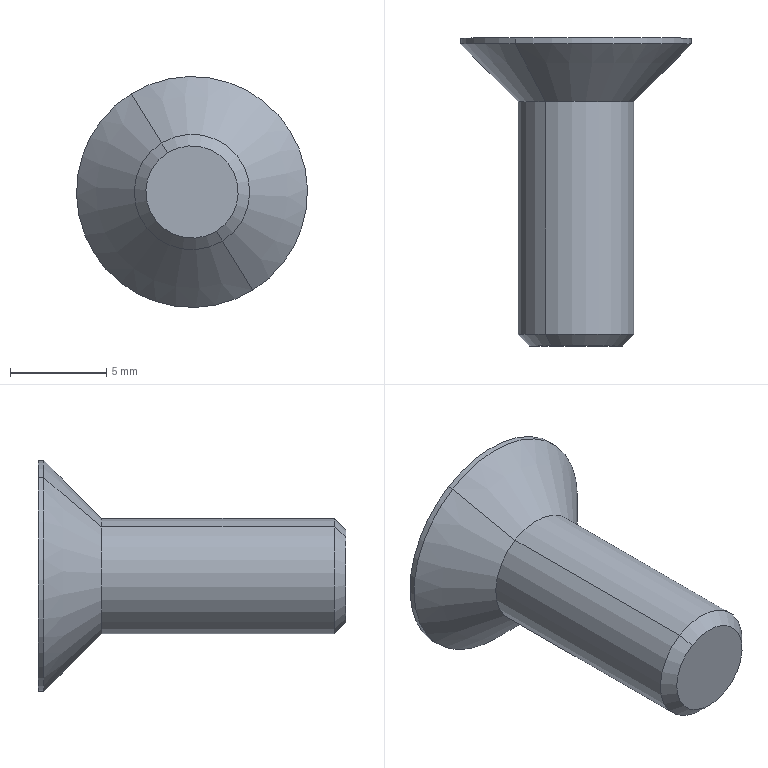Component | SolidWorks | 2012MB0201-1_UpperRackCoverModule-1_HexSocketFlatHeadScrewM6-16FerrousOxide-12 | 1 solid | 24 faces | box 12 x 16 x 12 mm | volume 549 mm3 | plane 14 | cone 6 | cylinder 4 | commonest cylinder face diameters 6 x2 12 x2 | material SCM435
STEP:
#1=COLOUR_RGB('',0.7922,0.8196,0.9333);
#2=FILL_AREA_STYLE_COLOUR('',#1);
#3=FILL_AREA_STYLE('',(#2));
#4=SURFACE_STYLE_FILL_AREA(#3);
#5=SURFACE_SIDE_STYLE('',(#4));
#6=SURFACE_STYLE_USAGE(.BOTH.,#5);
#7=PRESENTATION_STYLE_ASSIGNMENT((#6));
#8=CARTESIAN_POINT('',(-69.541,40.663,-12.118));
#9=VERTEX_POINT('',#8);
#10=CARTESIAN_POINT('',(-69.441,40.663,-12.278));
#11=VERTEX_POINT('',#10);
#12=CARTESIAN_POINT('',(-69.491,40.663,-12.198));
#13=DIRECTION('',(0.,-1.,-0.));
#14=DIRECTION('',(0.8493,0.,0.5279));
#15=AXIS2_PLACEMENT_3D('',#12,#13,#14);
#16=CIRCLE('',#15,0.09449);
#17=EDGE_CURVE('',#9,#11,#16,.T.);
#18=ORIENTED_EDGE('',*,*,#17,.F.);
#19=CARTESIAN_POINT('',(-69.553,40.687,-12.097));
#20=VERTEX_POINT('',#19);
#21=CARTESIAN_POINT('',(-69.541,40.663,-12.118));
#22=DIRECTION('',(-0.3733,0.7071,0.6005));
#23=VECTOR('',#22,39.37);
#24=LINE('',#21,#23);
#25=EDGE_CURVE('',#9,#20,#24,.T.);
#26=ORIENTED_EDGE('',*,*,#25,.T.);
#27=CARTESIAN_POINT('',(-69.429,40.687,-12.298));
#28=VERTEX_POINT('',#27);
#29=CARTESIAN_POINT('',(-69.491,40.687,-12.198));
#30=DIRECTION('',(-0.,1.,0.));
#31=DIRECTION('',(0.5279,0.,-0.8493));
#32=AXIS2_PLACEMENT_3D('',#29,#30,#31);
#33=CIRCLE('',#32,0.1181);
#34=EDGE_CURVE('',#28,#20,#33,.T.);
#35=ORIENTED_EDGE('',*,*,#34,.F.);
#36=CARTESIAN_POINT('',(-69.441,40.663,-12.278));
#37=DIRECTION('',(0.3733,0.7071,-0.6005));
#38=VECTOR('',#37,39.37);
#39=LINE('',#36,#38);
#40=EDGE_CURVE('',#11,#28,#39,.T.);
#41=ORIENTED_EDGE('',*,*,#40,.F.);
#42=EDGE_LOOP('',(#18,#26,#35,#41));
#43=FACE_OUTER_BOUND('',#42,.T.);
#44=CARTESIAN_POINT('',(-69.491,40.663,-12.198));
#45=DIRECTION('',(-0.,1.,0.));
#46=DIRECTION('',(0.5279,0.,-0.8493));
#47=AXIS2_PLACEMENT_3D('',#44,#45,#46);
#48=CONICAL_SURFACE('',#47,0.09449,0.7854);
#49=ADVANCED_FACE('',(#43),#48,.T.);
#50=ORIENTED_EDGE('',*,*,#34,.T.);
#51=CARTESIAN_POINT('',(-69.553,41.163,-12.097));
#52=VERTEX_POINT('',#51);
#53=CARTESIAN_POINT('',(-69.553,39.719,-12.097));
#54=DIRECTION('',(-0.,1.,0.));
#55=VECTOR('',#54,39.37);
#56=LINE('',#53,#55);
#57=EDGE_CURVE('',#20,#52,#56,.T.);
#58=ORIENTED_EDGE('',*,*,#57,.T.);
#59=CARTESIAN_POINT('',(-69.429,41.163,-12.298));
#60=VERTEX_POINT('',#59);
#61=CARTESIAN_POINT('',(-69.491,41.163,-12.198));
#62=DIRECTION('',(0.,-1.,-0.));
#63=DIRECTION('',(0.5279,0.,-0.8493));
#64=AXIS2_PLACEMENT_3D('',#61,#62,#63);
#65=CIRCLE('',#64,0.1181);
#66=EDGE_CURVE('',#52,#60,#65,.T.);
#67=ORIENTED_EDGE('',*,*,#66,.T.);
#68=CARTESIAN_POINT('',(-69.429,39.719,-12.298));
#69=DIRECTION('',(-0.,1.,0.));
#70=VECTOR('',#69,39.37);
#71=LINE('',#68,#70);
#72=EDGE_CURVE('',#28,#60,#71,.T.);
#73=ORIENTED_EDGE('',*,*,#72,.F.);
#74=EDGE_LOOP('',(#50,#58,#67,#73));
#75=FACE_OUTER_BOUND('',#74,.T.);
#76=CARTESIAN_POINT('',(-69.491,39.719,-12.198));
#77=DIRECTION('',(-0.,1.,0.));
#78=DIRECTION('',(0.5279,0.,-0.8493));
#79=AXIS2_PLACEMENT_3D('',#76,#77,#78);
#80=CYLINDRICAL_SURFACE('',#79,0.1181);
#81=ADVANCED_FACE('',(#75),#80,.T.);
#82=ORIENTED_EDGE('',*,*,#66,.F.);
#83=CARTESIAN_POINT('',(-69.616,41.282,-11.997));
#84=VERTEX_POINT('',#83);
#85=CARTESIAN_POINT('',(-69.616,41.282,-11.997));
#86=DIRECTION('',(-0.3733,0.7071,0.6005));
#87=VECTOR('',#86,39.37);
#88=LINE('',#85,#87);
#89=EDGE_CURVE('',#52,#84,#88,.T.);
#90=ORIENTED_EDGE('',*,*,#89,.T.);
#91=CARTESIAN_POINT('',(-69.366,41.282,-12.398));
#92=VERTEX_POINT('',#91);
#93=CARTESIAN_POINT('',(-69.491,41.282,-12.198));
#94=DIRECTION('',(0.,-1.,-0.));
#95=DIRECTION('',(0.5279,0.,-0.8493));
#96=AXIS2_PLACEMENT_3D('',#93,#94,#95);
#97=CIRCLE('',#96,0.2362);
#98=EDGE_CURVE('',#84,#92,#97,.T.);
#99=ORIENTED_EDGE('',*,*,#98,.T.);
#100=CARTESIAN_POINT('',(-69.366,41.282,-12.398));
#101=DIRECTION('',(0.3733,0.7071,-0.6005));
#102=VECTOR('',#101,39.37);
#103=LINE('',#100,#102);
#104=EDGE_CURVE('',#60,#92,#103,.T.);
#105=ORIENTED_EDGE('',*,*,#104,.F.);
#106=EDGE_LOOP('',(#82,#90,#99,#105));
#107=FACE_OUTER_BOUND('',#106,.T.);
#108=CARTESIAN_POINT('',(-69.491,41.282,-12.198));
#109=DIRECTION('',(-0.,1.,0.));
#110=DIRECTION('',(0.5279,0.,-0.8493));
#111=AXIS2_PLACEMENT_3D('',#108,#109,#110);
#112=CONICAL_SURFACE('',#111,0.2362,0.7854);
#113=ADVANCED_FACE('',(#107),#112,.T.);
#114=ORIENTED_EDGE('',*,*,#98,.F.);
#115=CARTESIAN_POINT('',(-69.616,41.293,-11.997));
#116=VERTEX_POINT('',#115);
#117=CARTESIAN_POINT('',(-69.616,39.719,-11.997));
#118=DIRECTION('',(-0.,1.,0.));
#119=VECTOR('',#118,39.37);
#120=LINE('',#117,#119);
#121=EDGE_CURVE('',#84,#116,#120,.T.);
#122=ORIENTED_EDGE('',*,*,#121,.T.);
#123=CARTESIAN_POINT('',(-69.366,41.293,-12.398));
#124=VERTEX_POINT('',#123);
#125=CARTESIAN_POINT('',(-69.491,41.293,-12.198));
#126=DIRECTION('',(0.,-1.,-0.));
#127=DIRECTION('',(0.5279,0.,-0.8493));
#128=AXIS2_PLACEMENT_3D('',#125,#126,#127);
#129=CIRCLE('',#128,0.2362);
#130=EDGE_CURVE('',#116,#124,#129,.T.);
#131=ORIENTED_EDGE('',*,*,#130,.T.);
#132=CARTESIAN_POINT('',(-69.366,39.719,-12.398));
#133=DIRECTION('',(-0.,1.,0.));
#134=VECTOR('',#133,39.37);
#135=LINE('',#132,#134);
#136=EDGE_CURVE('',#92,#124,#135,.T.);
#137=ORIENTED_EDGE('',*,*,#136,.F.);
#138=EDGE_LOOP('',(#114,#122,#131,#137));
#139=FACE_OUTER_BOUND('',#138,.T.);
#140=CARTESIAN_POINT('',(-69.491,39.719,-12.198));
#141=DIRECTION('',(-0.,1.,0.));
#142=DIRECTION('',(0.5279,0.,-0.8493));
#143=AXIS2_PLACEMENT_3D('',#140,#141,#142);
#144=CYLINDRICAL_SURFACE('',#143,0.2362);
#145=ADVANCED_FACE('',(#139),#144,.T.);
#146=CARTESIAN_POINT('',(-69.491,41.168,-12.198));
#147=VERTEX_POINT('',#146);
#148=CARTESIAN_POINT('',(-69.449,41.189,-12.265));
#149=VERTEX_POINT('',#148);
#150=CARTESIAN_POINT('',(-69.449,41.189,-12.265));
#151=DIRECTION('',(0.5099,0.2588,-0.8204));
#152=VECTOR('',#151,39.37);
#153=LINE('',#150,#152);
#154=EDGE_CURVE('',#147,#149,#153,.T.);
#155=ORIENTED_EDGE('',*,*,#154,.F.);
#156=CARTESIAN_POINT('',(-69.532,41.189,-12.131));
#157=VERTEX_POINT('',#156);
#158=CARTESIAN_POINT('',(-69.532,41.189,-12.131));
#159=DIRECTION('',(-0.5099,0.2588,0.8204));
#160=VECTOR('',#159,39.37);
#161=LINE('',#158,#160);
#162=EDGE_CURVE('',#147,#157,#161,.T.);
#163=ORIENTED_EDGE('',*,*,#162,.T.);
#164=CARTESIAN_POINT('',(-69.454,41.189,-12.128));
#165=VERTEX_POINT('',#164);
#166=CARTESIAN_POINT('',(-69.491,41.189,-12.198));
#167=DIRECTION('',(0.,-1.,-0.));
#168=DIRECTION('',(0.5279,0.,-0.8493));
#169=AXIS2_PLACEMENT_3D('',#166,#167,#168);
#170=CIRCLE('',#169,0.07874);
#171=EDGE_CURVE('',#165,#157,#170,.T.);
#172=ORIENTED_EDGE('',*,*,#171,.F.);
#173=CARTESIAN_POINT('',(-69.412,41.189,-12.195));
#174=VERTEX_POINT('',#173);
#175=CARTESIAN_POINT('',(-69.491,41.189,-12.198));
#176=DIRECTION('',(0.,-1.,-0.));
#177=DIRECTION('',(0.5279,0.,-0.8493));
#178=AXIS2_PLACEMENT_3D('',#175,#176,#177);
#179=CIRCLE('',#178,0.07874);
#180=EDGE_CURVE('',#174,#165,#179,.T.);
#181=ORIENTED_EDGE('',*,*,#180,.F.);
#182=CARTESIAN_POINT('',(-69.491,41.189,-12.198));
#183=DIRECTION('',(0.,-1.,-0.));
#184=DIRECTION('',(0.5279,0.,-0.8493));
#185=AXIS2_PLACEMENT_3D('',#182,#183,#184);
#186=CIRCLE('',#185,0.07874);
#187=EDGE_CURVE('',#149,#174,#186,.T.);
#188=ORIENTED_EDGE('',*,*,#187,.F.);
#189=EDGE_LOOP('',(#155,#163,#172,#181,#188));
#190=FACE_OUTER_BOUND('',#189,.T.);
#191=CARTESIAN_POINT('',(-69.491,41.189,-12.198));
#192=DIRECTION('',(-0.,1.,0.));
#193=DIRECTION('',(0.5279,0.,-0.8493));
#194=AXIS2_PLACEMENT_3D('',#191,#192,#193);
#195=CONICAL_SURFACE('',#194,0.07874,1.309);
#196=ADVANCED_FACE('',(#190),#195,.F.);
#197=ORIENTED_EDGE('',*,*,#57,.F.);
#198=CARTESIAN_POINT('',(-69.491,40.687,-12.198));
#199=DIRECTION('',(-0.,1.,0.));
#200=DIRECTION('',(0.5279,0.,-0.8493));
#201=AXIS2_PLACEMENT_3D('',#198,#199,#200);
#202=CIRCLE('',#201,0.1181);
#203=EDGE_CURVE('',#20,#28,#202,.T.);
#204=ORIENTED_EDGE('',*,*,#203,.T.);
#205=ORIENTED_EDGE('',*,*,#72,.T.);
#206=CARTESIAN_POINT('',(-69.491,41.163,-12.198));
#207=DIRECTION('',(0.,-1.,-0.));
#208=DIRECTION('',(0.5279,0.,-0.8493));
#209=AXIS2_PLACEMENT_3D('',#206,#207,#208);
#210=CIRCLE('',#209,0.1181);
#211=EDGE_CURVE('',#60,#52,#210,.T.);
#212=ORIENTED_EDGE('',*,*,#211,.T.);
#213=EDGE_LOOP('',(#197,#204,#205,#212));
#214=FACE_OUTER_BOUND('',#213,.T.);
#215=CARTESIAN_POINT('',(-69.491,39.719,-12.198));
#216=DIRECTION('',(-0.,1.,0.));
#217=DIRECTION('',(0.5279,0.,-0.8493));
#218=AXIS2_PLACEMENT_3D('',#215,#216,#217);
#219=CYLINDRICAL_SURFACE('',#218,0.1181);
#220=ADVANCED_FACE('',(#214),#219,.T.);
#221=ORIENTED_EDGE('',*,*,#89,.F.);
#222=ORIENTED_EDGE('',*,*,#211,.F.);
#223=ORIENTED_EDGE('',*,*,#104,.T.);
#224=CARTESIAN_POINT('',(-69.491,41.282,-12.198));
#225=DIRECTION('',(0.,-1.,-0.));
#226=DIRECTION('',(0.5279,0.,-0.8493));
#227=AXIS2_PLACEMENT_3D('',#224,#225,#226);
#228=CIRCLE('',#227,0.2362);
#229=EDGE_CURVE('',#92,#84,#228,.T.);
#230=ORIENTED_EDGE('',*,*,#229,.T.);
#231=EDGE_LOOP('',(#221,#222,#223,#230));
#232=FACE_OUTER_BOUND('',#231,.T.);
#233=CARTESIAN_POINT('',(-69.491,41.282,-12.198));
#234=DIRECTION('',(-0.,1.,0.));
#235=DIRECTION('',(0.5279,0.,-0.8493));
#236=AXIS2_PLACEMENT_3D('',#233,#234,#235);
#237=CONICAL_SURFACE('',#236,0.2362,0.7854);
#238=ADVANCED_FACE('',(#232),#237,.T.);
#239=ORIENTED_EDGE('',*,*,#121,.F.);
#240=ORIENTED_EDGE('',*,*,#229,.F.);
#241=ORIENTED_EDGE('',*,*,#136,.T.);
#242=CARTESIAN_POINT('',(-69.491,41.293,-12.198));
#243=DIRECTION('',(0.,-1.,-0.));
#244=DIRECTION('',(0.5279,0.,-0.8493));
#245=AXIS2_PLACEMENT_3D('',#242,#243,#244);
#246=CIRCLE('',#245,0.2362);
#247=EDGE_CURVE('',#124,#116,#246,.T.);
#248=ORIENTED_EDGE('',*,*,#247,.T.);
#249=EDGE_LOOP('',(#239,#240,#241,#248));
#250=FACE_OUTER_BOUND('',#249,.T.);
#251=CARTESIAN_POINT('',(-69.491,39.719,-12.198));
#252=DIRECTION('',(-0.,1.,0.));
#253=DIRECTION('',(0.5279,0.,-0.8493));
#254=AXIS2_PLACEMENT_3D('',#251,#252,#253);
#255=CYLINDRICAL_SURFACE('',#254,0.2362);
#256=ADVANCED_FACE('',(#250),#255,.T.);
#257=CARTESIAN_POINT('',(-69.494,41.293,-12.107));
#258=VERTEX_POINT('',#257);
#259=CARTESIAN_POINT('',(-69.414,41.293,-12.15));
#260=VERTEX_POINT('',#259);
#261=CARTESIAN_POINT('',(-69.494,41.293,-12.107));
#262=DIRECTION('',(0.8818,0.,-0.4716));
#263=VECTOR('',#262,39.37);
#264=LINE('',#261,#263);
#265=EDGE_CURVE('',#258,#260,#264,.T.);
#266=ORIENTED_EDGE('',*,*,#265,.F.);
#267=CARTESIAN_POINT('',(-69.571,41.293,-12.155));
#268=VERTEX_POINT('',#267);
#269=CARTESIAN_POINT('',(-69.532,41.293,-12.131));
#270=DIRECTION('',(0.8493,0.,0.5279));
#271=VECTOR('',#270,39.37);
#272=LINE('',#269,#271);
#273=EDGE_CURVE('',#268,#258,#272,.T.);
#274=ORIENTED_EDGE('',*,*,#273,.F.);
#275=CARTESIAN_POINT('',(-69.568,41.293,-12.246));
#276=VERTEX_POINT('',#275);
#277=CARTESIAN_POINT('',(-69.568,41.293,-12.246));
#278=DIRECTION('',(-0.03252,-0.,0.9995));
#279=VECTOR('',#278,39.37);
#280=LINE('',#277,#279);
#281=EDGE_CURVE('',#276,#268,#280,.T.);
#282=ORIENTED_EDGE('',*,*,#281,.F.);
#283=CARTESIAN_POINT('',(-69.488,41.293,-12.289));
#284=VERTEX_POINT('',#283);
#285=CARTESIAN_POINT('',(-69.488,41.293,-12.289));
#286=DIRECTION('',(-0.8818,-0.,0.4716));
#287=VECTOR('',#286,39.37);
#288=LINE('',#285,#287);
#289=EDGE_CURVE('',#284,#276,#288,.T.);
#290=ORIENTED_EDGE('',*,*,#289,.F.);
#291=CARTESIAN_POINT('',(-69.411,41.293,-12.241));
#292=VERTEX_POINT('',#291);
#293=CARTESIAN_POINT('',(-69.449,41.293,-12.265));
#294=DIRECTION('',(-0.8493,-0.,-0.5279));
#295=VECTOR('',#294,39.37);
#296=LINE('',#293,#295);
#297=EDGE_CURVE('',#292,#284,#296,.T.);
#298=ORIENTED_EDGE('',*,*,#297,.F.);
#299=CARTESIAN_POINT('',(-69.414,41.293,-12.15));
#300=DIRECTION('',(0.03252,0.,-0.9995));
#301=VECTOR('',#300,39.37);
#302=LINE('',#299,#301);
#303=EDGE_CURVE('',#260,#292,#302,.T.);
#304=ORIENTED_EDGE('',*,*,#303,.F.);
#305=EDGE_LOOP('',(#266,#274,#282,#290,#298,#304));
#306=FACE_BOUND('',#305,.T.);
#307=ORIENTED_EDGE('',*,*,#247,.F.);
#308=ORIENTED_EDGE('',*,*,#130,.F.);
#309=EDGE_LOOP('',(#307,#308));
#310=FACE_OUTER_BOUND('',#309,.T.);
#311=CARTESIAN_POINT('',(-69.491,41.293,-12.198));
#312=DIRECTION('',(0.,-1.,-0.));
#313=DIRECTION('',(-0.5279,-0.,0.8493));
#314=AXIS2_PLACEMENT_3D('',#311,#312,#313);
#315=PLANE('',#314);
#316=ADVANCED_FACE('',(#306,#310),#315,.F.);
#317=CARTESIAN_POINT('',(-69.414,41.189,-12.15));
#318=VERTEX_POINT('',#317);
#319=CARTESIAN_POINT('',(-69.412,41.189,-12.195));
#320=DIRECTION('',(-0.03252,-0.,0.9995));
#321=VECTOR('',#320,39.37);
#322=LINE('',#319,#321);
#323=EDGE_CURVE('',#174,#318,#322,.T.);
#324=ORIENTED_EDGE('',*,*,#323,.T.);
#325=CARTESIAN_POINT('',(-69.414,41.189,-12.15));
#326=DIRECTION('',(-0.,1.,0.));
#327=VECTOR('',#326,39.37);
#328=LINE('',#325,#327);
#329=EDGE_CURVE('',#318,#260,#328,.T.);
#330=ORIENTED_EDGE('',*,*,#329,.T.);
#331=ORIENTED_EDGE('',*,*,#303,.T.);
#332=CARTESIAN_POINT('',(-69.411,41.189,-12.241));
#333=VERTEX_POINT('',#332);
#334=CARTESIAN_POINT('',(-69.411,41.189,-12.241));
#335=DIRECTION('',(0.,-1.,-0.));
#336=VECTOR('',#335,39.37);
#337=LINE('',#334,#336);
#338=EDGE_CURVE('',#292,#333,#337,.T.);
#339=ORIENTED_EDGE('',*,*,#338,.T.);
#340=CARTESIAN_POINT('',(-69.411,41.189,-12.241));
#341=DIRECTION('',(-0.03252,-0.,0.9995));
#342=VECTOR('',#341,39.37);
#343=LINE('',#340,#342);
#344=EDGE_CURVE('',#333,#174,#343,.T.);
#345=ORIENTED_EDGE('',*,*,#344,.T.);
#346=EDGE_LOOP('',(#324,#330,#331,#339,#345));
#347=FACE_OUTER_BOUND('',#346,.T.);
#348=CARTESIAN_POINT('',(-69.411,41.189,-12.241));
#349=DIRECTION('',(-0.9995,-0.,-0.03252));
#350=DIRECTION('',(0.03252,0.,-0.9995));
#351=AXIS2_PLACEMENT_3D('',#348,#349,#350);
#352=PLANE('',#351);
#353=ADVANCED_FACE('',(#347),#352,.T.);
#354=CARTESIAN_POINT('',(-69.494,41.189,-12.107));
#355=VERTEX_POINT('',#354);
#356=CARTESIAN_POINT('',(-69.454,41.189,-12.128));
#357=DIRECTION('',(-0.8818,-0.,0.4716));
#358=VECTOR('',#357,39.37);
#359=LINE('',#356,#358);
#360=EDGE_CURVE('',#165,#355,#359,.T.);
#361=ORIENTED_EDGE('',*,*,#360,.T.);
#362=CARTESIAN_POINT('',(-69.494,41.189,-12.107));
#363=DIRECTION('',(-0.,1.,0.));
#364=VECTOR('',#363,39.37);
#365=LINE('',#362,#364);
#366=EDGE_CURVE('',#355,#258,#365,.T.);
#367=ORIENTED_EDGE('',*,*,#366,.T.);
#368=ORIENTED_EDGE('',*,*,#265,.T.);
#369=ORIENTED_EDGE('',*,*,#329,.F.);
#370=CARTESIAN_POINT('',(-69.414,41.189,-12.15));
#371=DIRECTION('',(-0.8818,-0.,0.4716));
#372=VECTOR('',#371,39.37);
#373=LINE('',#370,#372);
#374=EDGE_CURVE('',#318,#165,#373,.T.);
#375=ORIENTED_EDGE('',*,*,#374,.T.);
#376=EDGE_LOOP('',(#361,#367,#368,#369,#375));
#377=FACE_OUTER_BOUND('',#376,.T.);
#378=CARTESIAN_POINT('',(-69.414,41.189,-12.15));
#379=DIRECTION('',(-0.4716,-0.,-0.8818));
#380=DIRECTION('',(0.8818,0.,-0.4716));
#381=AXIS2_PLACEMENT_3D('',#378,#379,#380);
#382=PLANE('',#381);
#383=ADVANCED_FACE('',(#377),#382,.T.);
#384=CARTESIAN_POINT('',(-69.571,41.189,-12.155));
#385=VERTEX_POINT('',#384);
#386=CARTESIAN_POINT('',(-69.532,41.189,-12.131));
#387=DIRECTION('',(-0.8493,-0.,-0.5279));
#388=VECTOR('',#387,39.37);
#389=LINE('',#386,#388);
#390=EDGE_CURVE('',#157,#385,#389,.T.);
#391=ORIENTED_EDGE('',*,*,#390,.T.);
#392=CARTESIAN_POINT('',(-69.571,41.189,-12.155));
#393=DIRECTION('',(-0.,1.,0.));
#394=VECTOR('',#393,39.37);
#395=LINE('',#392,#394);
#396=EDGE_CURVE('',#385,#268,#395,.T.);
#397=ORIENTED_EDGE('',*,*,#396,.T.);
#398=ORIENTED_EDGE('',*,*,#273,.T.);
#399=ORIENTED_EDGE('',*,*,#366,.F.);
#400=CARTESIAN_POINT('',(-69.532,41.189,-12.131));
#401=DIRECTION('',(-0.8493,-0.,-0.5279));
#402=VECTOR('',#401,39.37);
#403=LINE('',#400,#402);
#404=EDGE_CURVE('',#355,#157,#403,.T.);
#405=ORIENTED_EDGE('',*,*,#404,.T.);
#406=EDGE_LOOP('',(#391,#397,#398,#399,#405));
#407=FACE_OUTER_BOUND('',#406,.T.);
#408=CARTESIAN_POINT('',(-69.494,41.189,-12.107));
#409=DIRECTION('',(0.5279,0.,-0.8493));
#410=DIRECTION('',(0.,-1.,-0.));
#411=AXIS2_PLACEMENT_3D('',#408,#409,#410);
#412=PLANE('',#411);
#413=ADVANCED_FACE('',(#407),#412,.T.);
#414=CARTESIAN_POINT('',(-69.57,41.189,-12.2));
#415=VERTEX_POINT('',#414);
#416=CARTESIAN_POINT('',(-69.568,41.189,-12.246));
#417=VERTEX_POINT('',#416);
#418=CARTESIAN_POINT('',(-69.57,41.189,-12.2));
#419=DIRECTION('',(0.03252,0.,-0.9995));
#420=VECTOR('',#419,39.37);
#421=LINE('',#418,#420);
#422=EDGE_CURVE('',#415,#417,#421,.T.);
#423=ORIENTED_EDGE('',*,*,#422,.T.);
#424=CARTESIAN_POINT('',(-69.568,41.189,-12.246));
#425=DIRECTION('',(-0.,1.,0.));
#426=VECTOR('',#425,39.37);
#427=LINE('',#424,#426);
#428=EDGE_CURVE('',#417,#276,#427,.T.);
#429=ORIENTED_EDGE('',*,*,#428,.T.);
#430=ORIENTED_EDGE('',*,*,#281,.T.);
#431=ORIENTED_EDGE('',*,*,#396,.F.);
#432=CARTESIAN_POINT('',(-69.571,41.189,-12.155));
#433=DIRECTION('',(0.03252,0.,-0.9995));
#434=VECTOR('',#433,39.37);
#435=LINE('',#432,#434);
#436=EDGE_CURVE('',#385,#415,#435,.T.);
#437=ORIENTED_EDGE('',*,*,#436,.T.);
#438=EDGE_LOOP('',(#423,#429,#430,#431,#437));
#439=FACE_OUTER_BOUND('',#438,.T.);
#440=CARTESIAN_POINT('',(-69.571,41.189,-12.155));
#441=DIRECTION('',(0.9995,0.,0.03252));
#442=DIRECTION('',(-0.03252,-0.,0.9995));
#443=AXIS2_PLACEMENT_3D('',#440,#441,#442);
#444=PLANE('',#443);
#445=ADVANCED_FACE('',(#439),#444,.T.);
#446=CARTESIAN_POINT('',(-69.528,41.189,-12.267));
#447=VERTEX_POINT('',#446);
#448=CARTESIAN_POINT('',(-69.488,41.189,-12.289));
#449=VERTEX_POINT('',#448);
#450=CARTESIAN_POINT('',(-69.568,41.189,-12.246));
#451=DIRECTION('',(0.8818,0.,-0.4716));
#452=VECTOR('',#451,39.37);
#453=LINE('',#450,#452);
#454=EDGE_CURVE('',#447,#449,#453,.T.);
#455=ORIENTED_EDGE('',*,*,#454,.T.);
#456=CARTESIAN_POINT('',(-69.488,41.189,-12.289));
#457=DIRECTION('',(-0.,1.,0.));
#458=VECTOR('',#457,39.37);
#459=LINE('',#456,#458);
#460=EDGE_CURVE('',#449,#284,#459,.T.);
#461=ORIENTED_EDGE('',*,*,#460,.T.);
#462=ORIENTED_EDGE('',*,*,#289,.T.);
#463=ORIENTED_EDGE('',*,*,#428,.F.);
#464=CARTESIAN_POINT('',(-69.568,41.189,-12.246));
#465=DIRECTION('',(0.8818,0.,-0.4716));
#466=VECTOR('',#465,39.37);
#467=LINE('',#464,#466);
#468=EDGE_CURVE('',#417,#447,#467,.T.);
#469=ORIENTED_EDGE('',*,*,#468,.T.);
#470=EDGE_LOOP('',(#455,#461,#462,#463,#469));
#471=FACE_OUTER_BOUND('',#470,.T.);
#472=CARTESIAN_POINT('',(-69.568,41.189,-12.246));
#473=DIRECTION('',(0.4716,0.,0.8818));
#474=DIRECTION('',(-0.8818,-0.,0.4716));
#475=AXIS2_PLACEMENT_3D('',#472,#473,#474);
#476=PLANE('',#475);
#477=ADVANCED_FACE('',(#471),#476,.T.);
#478=CARTESIAN_POINT('',(-69.449,41.189,-12.265));
#479=DIRECTION('',(0.8493,0.,0.5279));
#480=VECTOR('',#479,39.37);
#481=LINE('',#478,#480);
#482=EDGE_CURVE('',#149,#333,#481,.T.);
#483=ORIENTED_EDGE('',*,*,#482,.T.);
#484=ORIENTED_EDGE('',*,*,#338,.F.);
#485=ORIENTED_EDGE('',*,*,#297,.T.);
#486=ORIENTED_EDGE('',*,*,#460,.F.);
#487=CARTESIAN_POINT('',(-69.488,41.189,-12.289));
#488=DIRECTION('',(0.8493,0.,0.5279));
#489=VECTOR('',#488,39.37);
#490=LINE('',#487,#489);
#491=EDGE_CURVE('',#449,#149,#490,.T.);
#492=ORIENTED_EDGE('',*,*,#491,.T.);
#493=EDGE_LOOP('',(#483,#484,#485,#486,#492));
#494=FACE_OUTER_BOUND('',#493,.T.);
#495=CARTESIAN_POINT('',(-69.488,41.189,-12.289));
#496=DIRECTION('',(-0.5279,-0.,0.8493));
#497=DIRECTION('',(-0.,1.,0.));
#498=AXIS2_PLACEMENT_3D('',#495,#496,#497);
#499=PLANE('',#498);
#500=ADVANCED_FACE('',(#494),#499,.T.);
#501=ORIENTED_EDGE('',*,*,#491,.F.);
#502=ORIENTED_EDGE('',*,*,#454,.F.);
#503=CARTESIAN_POINT('',(-69.491,41.189,-12.198));
#504=DIRECTION('',(-0.,1.,0.));
#505=DIRECTION('',(0.5279,0.,-0.8493));
#506=AXIS2_PLACEMENT_3D('',#503,#504,#505);
#507=CIRCLE('',#506,0.07874);
#508=EDGE_CURVE('',#149,#447,#507,.T.);
#509=ORIENTED_EDGE('',*,*,#508,.F.);
#510=EDGE_LOOP('',(#501,#502,#509));
#511=FACE_OUTER_BOUND('',#510,.T.);
#512=CARTESIAN_POINT('',(-69.491,41.189,-12.198));
#513=DIRECTION('',(0.,-1.,-0.));
#514=DIRECTION('',(-0.5279,-0.,0.8493));
#515=AXIS2_PLACEMENT_3D('',#512,#513,#514);
#516=PLANE('',#515);
#517=ADVANCED_FACE('',(#511),#516,.F.);
#518=ORIENTED_EDGE('',*,*,#162,.F.);
#519=ORIENTED_EDGE('',*,*,#154,.T.);
#520=ORIENTED_EDGE('',*,*,#508,.T.);
#521=CARTESIAN_POINT('',(-69.491,41.189,-12.198));
#522=DIRECTION('',(0.,-1.,-0.));
#523=DIRECTION('',(0.5279,0.,-0.8493));
#524=AXIS2_PLACEMENT_3D('',#521,#522,#523);
#525=CIRCLE('',#524,0.07874);
#526=EDGE_CURVE('',#415,#447,#525,.T.);
#527=ORIENTED_EDGE('',*,*,#526,.F.);
#528=CARTESIAN_POINT('',(-69.491,41.189,-12.198));
#529=DIRECTION('',(0.,-1.,-0.));
#530=DIRECTION('',(0.5279,0.,-0.8493));
#531=AXIS2_PLACEMENT_3D('',#528,#529,#530);
#532=CIRCLE('',#531,0.07874);
#533=EDGE_CURVE('',#157,#415,#532,.T.);
#534=ORIENTED_EDGE('',*,*,#533,.F.);
#535=EDGE_LOOP('',(#518,#519,#520,#527,#534));
#536=FACE_OUTER_BOUND('',#535,.T.);
#537=CARTESIAN_POINT('',(-69.491,41.189,-12.198));
#538=DIRECTION('',(-0.,1.,0.));
#539=DIRECTION('',(0.5279,0.,-0.8493));
#540=AXIS2_PLACEMENT_3D('',#537,#538,#539);
#541=CONICAL_SURFACE('',#540,0.07874,1.309);
#542=ADVANCED_FACE('',(#536),#541,.F.);
#543=ORIENTED_EDGE('',*,*,#526,.T.);
#544=ORIENTED_EDGE('',*,*,#468,.F.);
#545=ORIENTED_EDGE('',*,*,#422,.F.);
#546=EDGE_LOOP('',(#543,#544,#545));
#547=FACE_OUTER_BOUND('',#546,.T.);
#548=CARTESIAN_POINT('',(-69.491,41.189,-12.198));
#549=DIRECTION('',(0.,-1.,-0.));
#550=DIRECTION('',(-0.5279,-0.,0.8493));
#551=AXIS2_PLACEMENT_3D('',#548,#549,#550);
#552=PLANE('',#551);
#553=ADVANCED_FACE('',(#547),#552,.F.);
#554=ORIENTED_EDGE('',*,*,#436,.F.);
#555=ORIENTED_EDGE('',*,*,#390,.F.);
#556=ORIENTED_EDGE('',*,*,#533,.T.);
#557=EDGE_LOOP('',(#554,#555,#556));
#558=FACE_OUTER_BOUND('',#557,.T.);
#559=CARTESIAN_POINT('',(-69.491,41.189,-12.198));
#560=DIRECTION('',(0.,-1.,-0.));
#561=DIRECTION('',(-0.5279,-0.,0.8493));
#562=AXIS2_PLACEMENT_3D('',#559,#560,#561);
#563=PLANE('',#562);
#564=ADVANCED_FACE('',(#558),#563,.F.);
#565=ORIENTED_EDGE('',*,*,#404,.F.);
#566=ORIENTED_EDGE('',*,*,#360,.F.);
#567=ORIENTED_EDGE('',*,*,#171,.T.);
#568=EDGE_LOOP('',(#565,#566,#567));
#569=FACE_OUTER_BOUND('',#568,.T.);
#570=CARTESIAN_POINT('',(-69.491,41.189,-12.198));
#571=DIRECTION('',(0.,-1.,-0.));
#572=DIRECTION('',(-0.5279,-0.,0.8493));
#573=AXIS2_PLACEMENT_3D('',#570,#571,#572);
#574=PLANE('',#573);
#575=ADVANCED_FACE('',(#569),#574,.F.);
#576=ORIENTED_EDGE('',*,*,#374,.F.);
#577=ORIENTED_EDGE('',*,*,#323,.F.);
#578=ORIENTED_EDGE('',*,*,#180,.T.);
#579=EDGE_LOOP('',(#576,#577,#578));
#580=FACE_OUTER_BOUND('',#579,.T.);
#581=CARTESIAN_POINT('',(-69.491,41.189,-12.198));
#582=DIRECTION('',(0.,-1.,-0.));
#583=DIRECTION('',(-0.5279,-0.,0.8493));
#584=AXIS2_PLACEMENT_3D('',#581,#582,#583);
#585=PLANE('',#584);
#586=ADVANCED_FACE('',(#580),#585,.F.);
#587=ORIENTED_EDGE('',*,*,#344,.F.);
#588=ORIENTED_EDGE('',*,*,#482,.F.);
#589=ORIENTED_EDGE('',*,*,#187,.T.);
#590=EDGE_LOOP('',(#587,#588,#589));
#591=FACE_OUTER_BOUND('',#590,.T.);
#592=CARTESIAN_POINT('',(-69.491,41.189,-12.198));
#593=DIRECTION('',(0.,-1.,-0.));
#594=DIRECTION('',(-0.5279,-0.,0.8493));
#595=AXIS2_PLACEMENT_3D('',#592,#593,#594);
#596=PLANE('',#595);
#597=ADVANCED_FACE('',(#591),#596,.F.);
#598=CARTESIAN_POINT('',(-69.491,40.663,-12.198));
#599=DIRECTION('',(0.,-1.,-0.));
#600=DIRECTION('',(0.8493,0.,0.5279));
#601=AXIS2_PLACEMENT_3D('',#598,#599,#600);
#602=CIRCLE('',#601,0.09449);
#603=EDGE_CURVE('',#11,#9,#602,.T.);
#604=ORIENTED_EDGE('',*,*,#603,.T.);
#605=ORIENTED_EDGE('',*,*,#17,.T.);
#606=EDGE_LOOP('',(#604,#605));
#607=FACE_OUTER_BOUND('',#606,.T.);
#608=CARTESIAN_POINT('',(-69.904,40.663,-12.223));
#609=DIRECTION('',(-0.,1.,0.));
#610=DIRECTION('',(0.8493,0.,0.5279));
#611=AXIS2_PLACEMENT_3D('',#608,#609,#610);
#612=PLANE('',#611);
#613=ADVANCED_FACE('',(#607),#612,.F.);
#614=ORIENTED_EDGE('',*,*,#25,.F.);
#615=ORIENTED_EDGE('',*,*,#603,.F.);
#616=ORIENTED_EDGE('',*,*,#40,.T.);
#617=ORIENTED_EDGE('',*,*,#203,.F.);
#618=EDGE_LOOP('',(#614,#615,#616,#617));
#619=FACE_OUTER_BOUND('',#618,.T.);
#620=CARTESIAN_POINT('',(-69.491,40.663,-12.198));
#621=DIRECTION('',(-0.,1.,0.));
#622=DIRECTION('',(0.5279,0.,-0.8493));
#623=AXIS2_PLACEMENT_3D('',#620,#621,#622);
#624=CONICAL_SURFACE('',#623,0.09449,0.7854);
#625=ADVANCED_FACE('',(#619),#624,.T.);
#626=CLOSED_SHELL('',(#49,#81,#113,#145,#196,#220,#238,#256,#316,#353,#383,#413,#445,#477,#500,#517,#542,#553,#564,#575,#586,#597,#613,#625));
#627=MANIFOLD_SOLID_BREP('',#626);
#628=STYLED_ITEM('',(#7),#627);
#629=PRESENTATION_LAYER_ASSIGNMENT('','',(#628));
#630=(LENGTH_UNIT()NAMED_UNIT(*)SI_UNIT($,.METRE.));
#631=LENGTH_MEASURE_WITH_UNIT(LENGTH_MEASURE(0.0254),#630);
#632=DIMENSIONAL_EXPONENTS(1.,0.,0.,0.,0.,0.,0.);
#633=(CONVERSION_BASED_UNIT('',#631)LENGTH_UNIT()NAMED_UNIT(#632));
#634=UNCERTAINTY_MEASURE_WITH_UNIT(LENGTH_MEASURE(0.00001),#633,'','');
#635=(NAMED_UNIT(*)PLANE_ANGLE_UNIT()SI_UNIT($,.RADIAN.));
#636=(NAMED_UNIT(*)SI_UNIT($,.STERADIAN.)SOLID_ANGLE_UNIT());
#637=(GEOMETRIC_REPRESENTATION_CONTEXT(3)GLOBAL_UNCERTAINTY_ASSIGNED_CONTEXT((#634))GLOBAL_UNIT_ASSIGNED_CONTEXT((#633,#635,#636))REPRESENTATION_CONTEXT('',''));
#638=MECHANICAL_DESIGN_GEOMETRIC_PRESENTATION_REPRESENTATION('',(#628),#637);
#639=CARTESIAN_POINT('',(0.,0.,0.));
#640=DIRECTION('',(0.,0.,1.));
#641=DIRECTION('',(1.,0.,0.));
#642=AXIS2_PLACEMENT_3D('',#639,#640,#641);
#643=(LENGTH_UNIT()NAMED_UNIT(*)SI_UNIT($,.METRE.));
#644=LENGTH_MEASURE_WITH_UNIT(LENGTH_MEASURE(0.0254),#643);
#645=DIMENSIONAL_EXPONENTS(1.,0.,0.,0.,0.,0.,0.);
#646=(CONVERSION_BASED_UNIT('',#644)LENGTH_UNIT()NAMED_UNIT(#645));
#647=UNCERTAINTY_MEASURE_WITH_UNIT(LENGTH_MEASURE(0.00001),#646,'','');
#648=(NAMED_UNIT(*)PLANE_ANGLE_UNIT()SI_UNIT($,.RADIAN.));
#649=(NAMED_UNIT(*)SI_UNIT($,.STERADIAN.)SOLID_ANGLE_UNIT());
#650=(GEOMETRIC_REPRESENTATION_CONTEXT(3)GLOBAL_UNCERTAINTY_ASSIGNED_CONTEXT((#647))GLOBAL_UNIT_ASSIGNED_CONTEXT((#646,#648,#649))REPRESENTATION_CONTEXT('',''));
#651=ADVANCED_BREP_SHAPE_REPRESENTATION('',(#627,#642),#650);